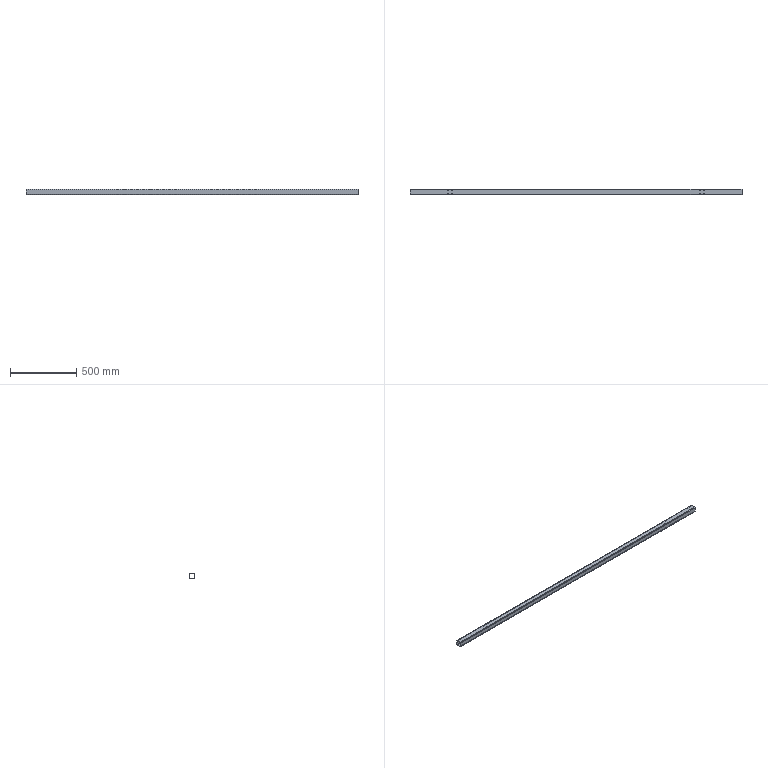Component | NX | LONG_BOT_ROD | 1 solid | 42 faces | volume 1108695 mm3 | cylinder 32 | plane 10 | commonest cylinder face diameters 8 x16 5 x8 6 x8